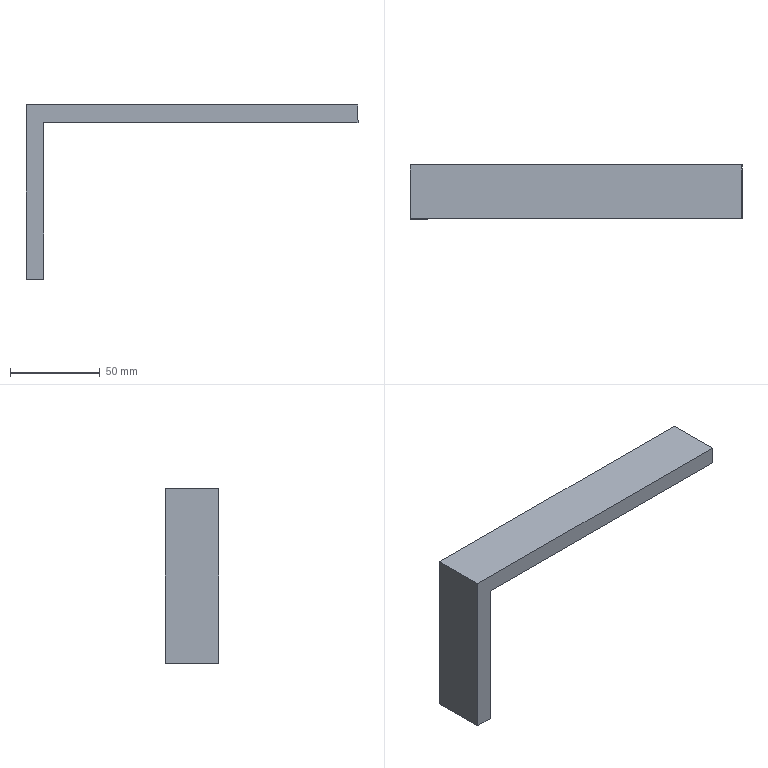Component | SolidWorks | OuterBagStorageAssembly-1_Copy_of_Part22-1 | 1 solid | 8 faces | box 185 x 30 x 97 mm | volume 81600 mm3 | plane 8
build123d program:
from build123d import *

# Parameters (mm, degrees)
BOSS_EXTRUDE1_DEPTH = 30


with BuildPart() as part:
    # Sketch2 → Boss-Extrude1 (new body)
    with BuildSketch(Plane.XY):
        Polygon((-141.073, -118.121), (-44.073, -118.121), (-44.073, 66.879), (-54.073, 66.879), (-54.073, -108.121), (-141.073, -108.121), align=None)
    extrude(amount=-BOSS_EXTRUDE1_DEPTH)


solid = part.part

# Placed as in the assembly
solid = solid.moved(Location((-315.175, 257.349, 386.24), (-90, 0, -90)))
STEP:
#1=COLOUR_RGB('',0.7922,0.8196,0.9333);
#2=FILL_AREA_STYLE_COLOUR('',#1);
#3=FILL_AREA_STYLE('',(#2));
#4=SURFACE_STYLE_FILL_AREA(#3);
#5=SURFACE_SIDE_STYLE('',(#4));
#6=SURFACE_STYLE_USAGE(.BOTH.,#5);
#7=PRESENTATION_STYLE_ASSIGNMENT((#6));
#8=CARTESIAN_POINT('',(-16.665,10.132,9.652));
#9=VERTEX_POINT('',#8);
#10=CARTESIAN_POINT('',(-17.059,10.132,9.652));
#11=VERTEX_POINT('',#10);
#12=CARTESIAN_POINT('',(-17.059,10.132,9.652));
#13=DIRECTION('',(-1.,0.,-0.));
#14=VECTOR('',#13,39.37);
#15=LINE('',#12,#14);
#16=EDGE_CURVE('',#9,#11,#15,.T.);
#17=ORIENTED_EDGE('',*,*,#16,.F.);
#18=CARTESIAN_POINT('',(-16.665,8.951,9.652));
#19=VERTEX_POINT('',#18);
#20=CARTESIAN_POINT('',(-16.665,8.951,9.652));
#21=DIRECTION('',(0.,1.,-0.));
#22=VECTOR('',#21,39.37);
#23=LINE('',#20,#22);
#24=EDGE_CURVE('',#19,#9,#23,.T.);
#25=ORIENTED_EDGE('',*,*,#24,.F.);
#26=CARTESIAN_POINT('',(-17.059,8.951,9.652));
#27=VERTEX_POINT('',#26);
#28=CARTESIAN_POINT('',(-17.059,8.951,9.652));
#29=DIRECTION('',(-1.,0.,-0.));
#30=VECTOR('',#29,39.37);
#31=LINE('',#28,#30);
#32=EDGE_CURVE('',#19,#27,#31,.T.);
#33=ORIENTED_EDGE('',*,*,#32,.T.);
#34=CARTESIAN_POINT('',(-17.059,8.951,9.652));
#35=DIRECTION('',(0.,1.,-0.));
#36=VECTOR('',#35,39.37);
#37=LINE('',#34,#36);
#38=EDGE_CURVE('',#27,#11,#37,.T.);
#39=ORIENTED_EDGE('',*,*,#38,.T.);
#40=EDGE_LOOP('',(#17,#25,#33,#39));
#41=FACE_OUTER_BOUND('',#40,.T.);
#42=CARTESIAN_POINT('',(-17.059,8.951,9.652));
#43=DIRECTION('',(0.,-0.,-1.));
#44=DIRECTION('',(0.,1.,-0.));
#45=AXIS2_PLACEMENT_3D('',#42,#43,#44);
#46=PLANE('',#45);
#47=ADVANCED_FACE('',(#41),#46,.T.);
#48=CARTESIAN_POINT('',(-16.665,10.132,13.077));
#49=VERTEX_POINT('',#48);
#50=CARTESIAN_POINT('',(-16.665,10.132,9.652));
#51=DIRECTION('',(0.,-0.,-1.));
#52=VECTOR('',#51,39.37);
#53=LINE('',#50,#52);
#54=EDGE_CURVE('',#49,#9,#53,.T.);
#55=ORIENTED_EDGE('',*,*,#54,.F.);
#56=CARTESIAN_POINT('',(-16.665,8.951,13.077));
#57=VERTEX_POINT('',#56);
#58=CARTESIAN_POINT('',(-16.665,8.951,13.077));
#59=DIRECTION('',(0.,1.,-0.));
#60=VECTOR('',#59,39.37);
#61=LINE('',#58,#60);
#62=EDGE_CURVE('',#57,#49,#61,.T.);
#63=ORIENTED_EDGE('',*,*,#62,.F.);
#64=CARTESIAN_POINT('',(-16.665,8.951,9.652));
#65=DIRECTION('',(0.,-0.,-1.));
#66=VECTOR('',#65,39.37);
#67=LINE('',#64,#66);
#68=EDGE_CURVE('',#57,#19,#67,.T.);
#69=ORIENTED_EDGE('',*,*,#68,.T.);
#70=ORIENTED_EDGE('',*,*,#24,.T.);
#71=EDGE_LOOP('',(#55,#63,#69,#70));
#72=FACE_OUTER_BOUND('',#71,.T.);
#73=CARTESIAN_POINT('',(-16.665,8.951,9.652));
#74=DIRECTION('',(1.,-0.,0.));
#75=DIRECTION('',(0.,1.,-0.));
#76=AXIS2_PLACEMENT_3D('',#73,#74,#75);
#77=PLANE('',#76);
#78=ADVANCED_FACE('',(#72),#77,.T.);
#79=CARTESIAN_POINT('',(-9.775,10.132,13.077));
#80=VERTEX_POINT('',#79);
#81=CARTESIAN_POINT('',(-16.665,10.132,13.077));
#82=DIRECTION('',(-1.,0.,-0.));
#83=VECTOR('',#82,39.37);
#84=LINE('',#81,#83);
#85=EDGE_CURVE('',#80,#49,#84,.T.);
#86=ORIENTED_EDGE('',*,*,#85,.F.);
#87=CARTESIAN_POINT('',(-9.775,8.951,13.077));
#88=VERTEX_POINT('',#87);
#89=CARTESIAN_POINT('',(-9.775,8.951,13.077));
#90=DIRECTION('',(0.,1.,-0.));
#91=VECTOR('',#90,39.37);
#92=LINE('',#89,#91);
#93=EDGE_CURVE('',#88,#80,#92,.T.);
#94=ORIENTED_EDGE('',*,*,#93,.F.);
#95=CARTESIAN_POINT('',(-16.665,8.951,13.077));
#96=DIRECTION('',(-1.,0.,-0.));
#97=VECTOR('',#96,39.37);
#98=LINE('',#95,#97);
#99=EDGE_CURVE('',#88,#57,#98,.T.);
#100=ORIENTED_EDGE('',*,*,#99,.T.);
#101=ORIENTED_EDGE('',*,*,#62,.T.);
#102=EDGE_LOOP('',(#86,#94,#100,#101));
#103=FACE_OUTER_BOUND('',#102,.T.);
#104=CARTESIAN_POINT('',(-16.665,8.951,13.077));
#105=DIRECTION('',(0.,-0.,-1.));
#106=DIRECTION('',(0.,1.,-0.));
#107=AXIS2_PLACEMENT_3D('',#104,#105,#106);
#108=PLANE('',#107);
#109=ADVANCED_FACE('',(#103),#108,.T.);
#110=CARTESIAN_POINT('',(-9.775,10.132,13.471));
#111=VERTEX_POINT('',#110);
#112=CARTESIAN_POINT('',(-9.775,10.132,13.471));
#113=DIRECTION('',(0.,-0.,-1.));
#114=VECTOR('',#113,39.37);
#115=LINE('',#112,#114);
#116=EDGE_CURVE('',#111,#80,#115,.T.);
#117=ORIENTED_EDGE('',*,*,#116,.F.);
#118=CARTESIAN_POINT('',(-9.775,8.951,13.471));
#119=VERTEX_POINT('',#118);
#120=CARTESIAN_POINT('',(-9.775,8.951,13.471));
#121=DIRECTION('',(0.,1.,-0.));
#122=VECTOR('',#121,39.37);
#123=LINE('',#120,#122);
#124=EDGE_CURVE('',#119,#111,#123,.T.);
#125=ORIENTED_EDGE('',*,*,#124,.F.);
#126=CARTESIAN_POINT('',(-9.775,8.951,13.471));
#127=DIRECTION('',(0.,-0.,-1.));
#128=VECTOR('',#127,39.37);
#129=LINE('',#126,#128);
#130=EDGE_CURVE('',#119,#88,#129,.T.);
#131=ORIENTED_EDGE('',*,*,#130,.T.);
#132=ORIENTED_EDGE('',*,*,#93,.T.);
#133=EDGE_LOOP('',(#117,#125,#131,#132));
#134=FACE_OUTER_BOUND('',#133,.T.);
#135=CARTESIAN_POINT('',(-9.775,8.951,13.471));
#136=DIRECTION('',(1.,-0.,0.));
#137=DIRECTION('',(0.,1.,-0.));
#138=AXIS2_PLACEMENT_3D('',#135,#136,#137);
#139=PLANE('',#138);
#140=ADVANCED_FACE('',(#134),#139,.T.);
#141=CARTESIAN_POINT('',(-17.059,10.132,13.471));
#142=VERTEX_POINT('',#141);
#143=CARTESIAN_POINT('',(-17.059,10.132,13.471));
#144=DIRECTION('',(1.,-0.,0.));
#145=VECTOR('',#144,39.37);
#146=LINE('',#143,#145);
#147=EDGE_CURVE('',#142,#111,#146,.T.);
#148=ORIENTED_EDGE('',*,*,#147,.F.);
#149=CARTESIAN_POINT('',(-17.059,8.951,13.471));
#150=VERTEX_POINT('',#149);
#151=CARTESIAN_POINT('',(-17.059,8.951,13.471));
#152=DIRECTION('',(0.,1.,-0.));
#153=VECTOR('',#152,39.37);
#154=LINE('',#151,#153);
#155=EDGE_CURVE('',#150,#142,#154,.T.);
#156=ORIENTED_EDGE('',*,*,#155,.F.);
#157=CARTESIAN_POINT('',(-17.059,8.951,13.471));
#158=DIRECTION('',(1.,-0.,0.));
#159=VECTOR('',#158,39.37);
#160=LINE('',#157,#159);
#161=EDGE_CURVE('',#150,#119,#160,.T.);
#162=ORIENTED_EDGE('',*,*,#161,.T.);
#163=ORIENTED_EDGE('',*,*,#124,.T.);
#164=EDGE_LOOP('',(#148,#156,#162,#163));
#165=FACE_OUTER_BOUND('',#164,.T.);
#166=CARTESIAN_POINT('',(-17.059,8.951,13.471));
#167=DIRECTION('',(-0.,0.,1.));
#168=DIRECTION('',(1.,-0.,0.));
#169=AXIS2_PLACEMENT_3D('',#166,#167,#168);
#170=PLANE('',#169);
#171=ADVANCED_FACE('',(#165),#170,.T.);
#172=CARTESIAN_POINT('',(-17.059,10.132,9.652));
#173=DIRECTION('',(-0.,0.,1.));
#174=VECTOR('',#173,39.37);
#175=LINE('',#172,#174);
#176=EDGE_CURVE('',#11,#142,#175,.T.);
#177=ORIENTED_EDGE('',*,*,#176,.F.);
#178=ORIENTED_EDGE('',*,*,#38,.F.);
#179=CARTESIAN_POINT('',(-17.059,8.951,9.652));
#180=DIRECTION('',(-0.,0.,1.));
#181=VECTOR('',#180,39.37);
#182=LINE('',#179,#181);
#183=EDGE_CURVE('',#27,#150,#182,.T.);
#184=ORIENTED_EDGE('',*,*,#183,.T.);
#185=ORIENTED_EDGE('',*,*,#155,.T.);
#186=EDGE_LOOP('',(#177,#178,#184,#185));
#187=FACE_OUTER_BOUND('',#186,.T.);
#188=CARTESIAN_POINT('',(-17.059,8.951,9.652));
#189=DIRECTION('',(-1.,0.,-0.));
#190=DIRECTION('',(-0.,-1.,0.));
#191=AXIS2_PLACEMENT_3D('',#188,#189,#190);
#192=PLANE('',#191);
#193=ADVANCED_FACE('',(#187),#192,.T.);
#194=ORIENTED_EDGE('',*,*,#32,.F.);
#195=ORIENTED_EDGE('',*,*,#68,.F.);
#196=ORIENTED_EDGE('',*,*,#99,.F.);
#197=ORIENTED_EDGE('',*,*,#130,.F.);
#198=ORIENTED_EDGE('',*,*,#161,.F.);
#199=ORIENTED_EDGE('',*,*,#183,.F.);
#200=EDGE_LOOP('',(#194,#195,#196,#197,#198,#199));
#201=FACE_OUTER_BOUND('',#200,.T.);
#202=CARTESIAN_POINT('',(-12.408,8.951,15.206));
#203=DIRECTION('',(-0.,-1.,0.));
#204=DIRECTION('',(0.,-0.,-1.));
#205=AXIS2_PLACEMENT_3D('',#202,#203,#204);
#206=PLANE('',#205);
#207=ADVANCED_FACE('',(#201),#206,.T.);
#208=ORIENTED_EDGE('',*,*,#16,.T.);
#209=ORIENTED_EDGE('',*,*,#176,.T.);
#210=ORIENTED_EDGE('',*,*,#147,.T.);
#211=ORIENTED_EDGE('',*,*,#116,.T.);
#212=ORIENTED_EDGE('',*,*,#85,.T.);
#213=ORIENTED_EDGE('',*,*,#54,.T.);
#214=EDGE_LOOP('',(#208,#209,#210,#211,#212,#213));
#215=FACE_OUTER_BOUND('',#214,.T.);
#216=CARTESIAN_POINT('',(-12.408,10.132,15.206));
#217=DIRECTION('',(-0.,-1.,0.));
#218=DIRECTION('',(0.,-0.,-1.));
#219=AXIS2_PLACEMENT_3D('',#216,#217,#218);
#220=PLANE('',#219);
#221=ADVANCED_FACE('',(#215),#220,.F.);
#222=CLOSED_SHELL('',(#47,#78,#109,#140,#171,#193,#207,#221));
#223=MANIFOLD_SOLID_BREP('',#222);
#224=STYLED_ITEM('',(#7),#223);
#225=PRESENTATION_LAYER_ASSIGNMENT('','',(#224));
#226=CARTESIAN_POINT('',(0.,0.,0.));
#227=DIRECTION('',(0.,0.,1.));
#228=DIRECTION('',(1.,0.,0.));
#229=AXIS2_PLACEMENT_3D('',#226,#227,#228);
#230=(LENGTH_UNIT()NAMED_UNIT(*)SI_UNIT($,.METRE.));
#231=LENGTH_MEASURE_WITH_UNIT(LENGTH_MEASURE(0.0254),#230);
#232=DIMENSIONAL_EXPONENTS(1.,0.,0.,0.,0.,0.,0.);
#233=(CONVERSION_BASED_UNIT('',#231)LENGTH_UNIT()NAMED_UNIT(#232));
#234=UNCERTAINTY_MEASURE_WITH_UNIT(LENGTH_MEASURE(0.00001),#233,'','');
#235=(NAMED_UNIT(*)PLANE_ANGLE_UNIT()SI_UNIT($,.RADIAN.));
#236=(NAMED_UNIT(*)SI_UNIT($,.STERADIAN.)SOLID_ANGLE_UNIT());
#237=(GEOMETRIC_REPRESENTATION_CONTEXT(3)GLOBAL_UNCERTAINTY_ASSIGNED_CONTEXT((#234))GLOBAL_UNIT_ASSIGNED_CONTEXT((#233,#235,#236))REPRESENTATION_CONTEXT('',''));
#238=ADVANCED_BREP_SHAPE_REPRESENTATION('',(#223,#229),#237);
#239=(LENGTH_UNIT()NAMED_UNIT(*)SI_UNIT($,.METRE.));
#240=LENGTH_MEASURE_WITH_UNIT(LENGTH_MEASURE(0.0254),#239);
#241=DIMENSIONAL_EXPONENTS(1.,0.,0.,0.,0.,0.,0.);
#242=(CONVERSION_BASED_UNIT('',#240)LENGTH_UNIT()NAMED_UNIT(#241));
#243=UNCERTAINTY_MEASURE_WITH_UNIT(LENGTH_MEASURE(0.00001),#242,'','');
#244=(NAMED_UNIT(*)PLANE_ANGLE_UNIT()SI_UNIT($,.RADIAN.));
#245=(NAMED_UNIT(*)SI_UNIT($,.STERADIAN.)SOLID_ANGLE_UNIT());
#246=(GEOMETRIC_REPRESENTATION_CONTEXT(3)GLOBAL_UNCERTAINTY_ASSIGNED_CONTEXT((#243))GLOBAL_UNIT_ASSIGNED_CONTEXT((#242,#244,#245))REPRESENTATION_CONTEXT('',''));
#247=MECHANICAL_DESIGN_GEOMETRIC_PRESENTATION_REPRESENTATION('',(#224),#246);